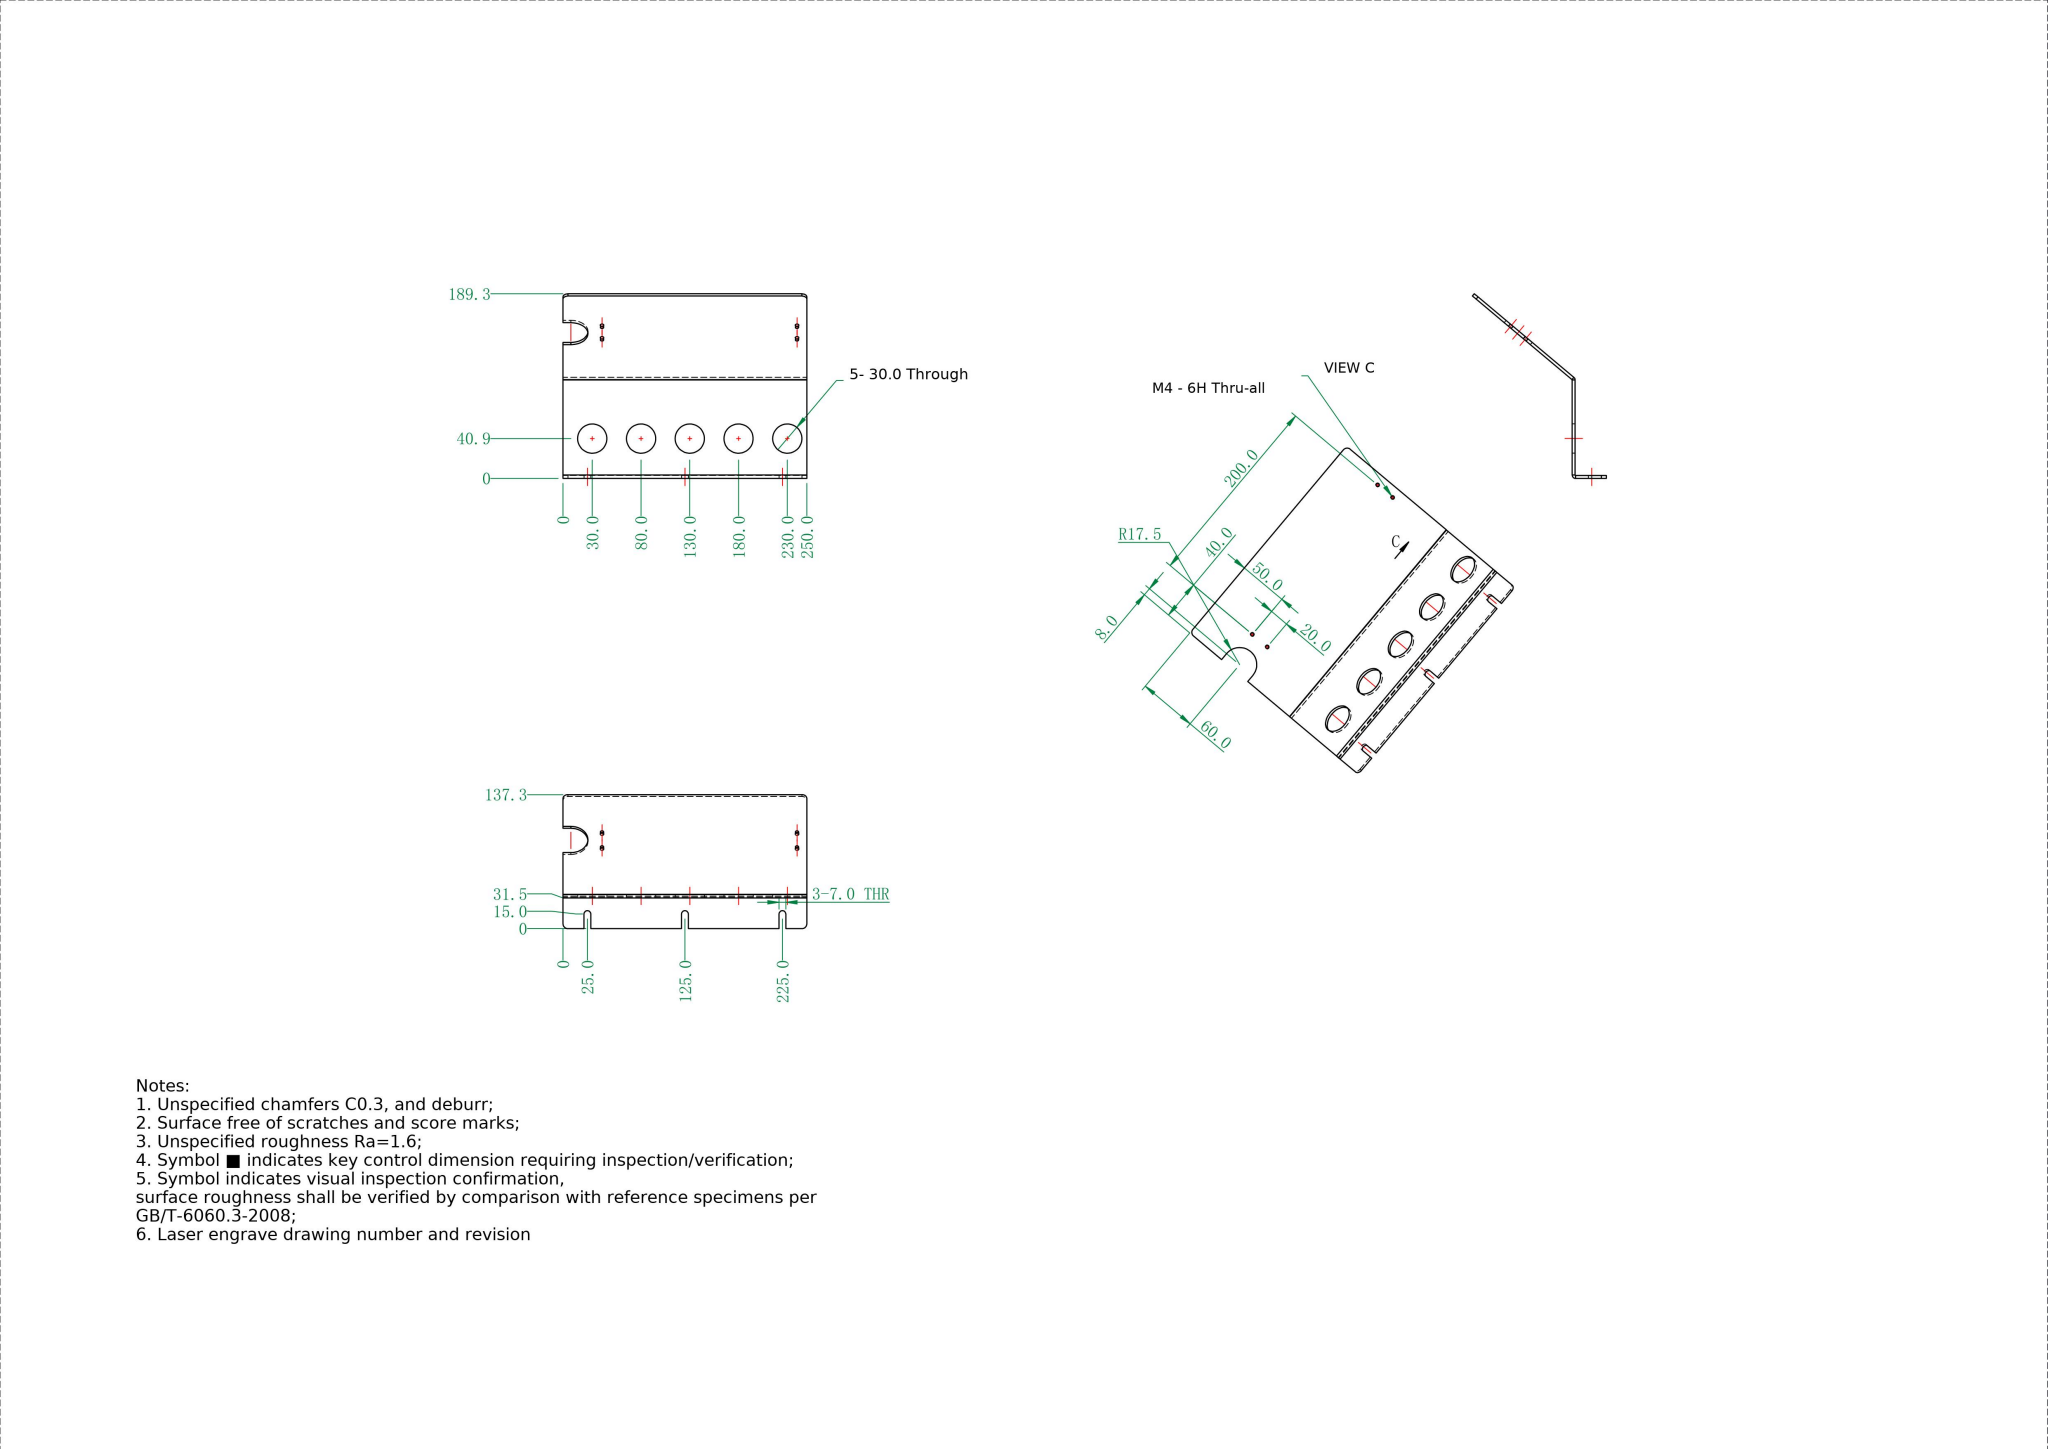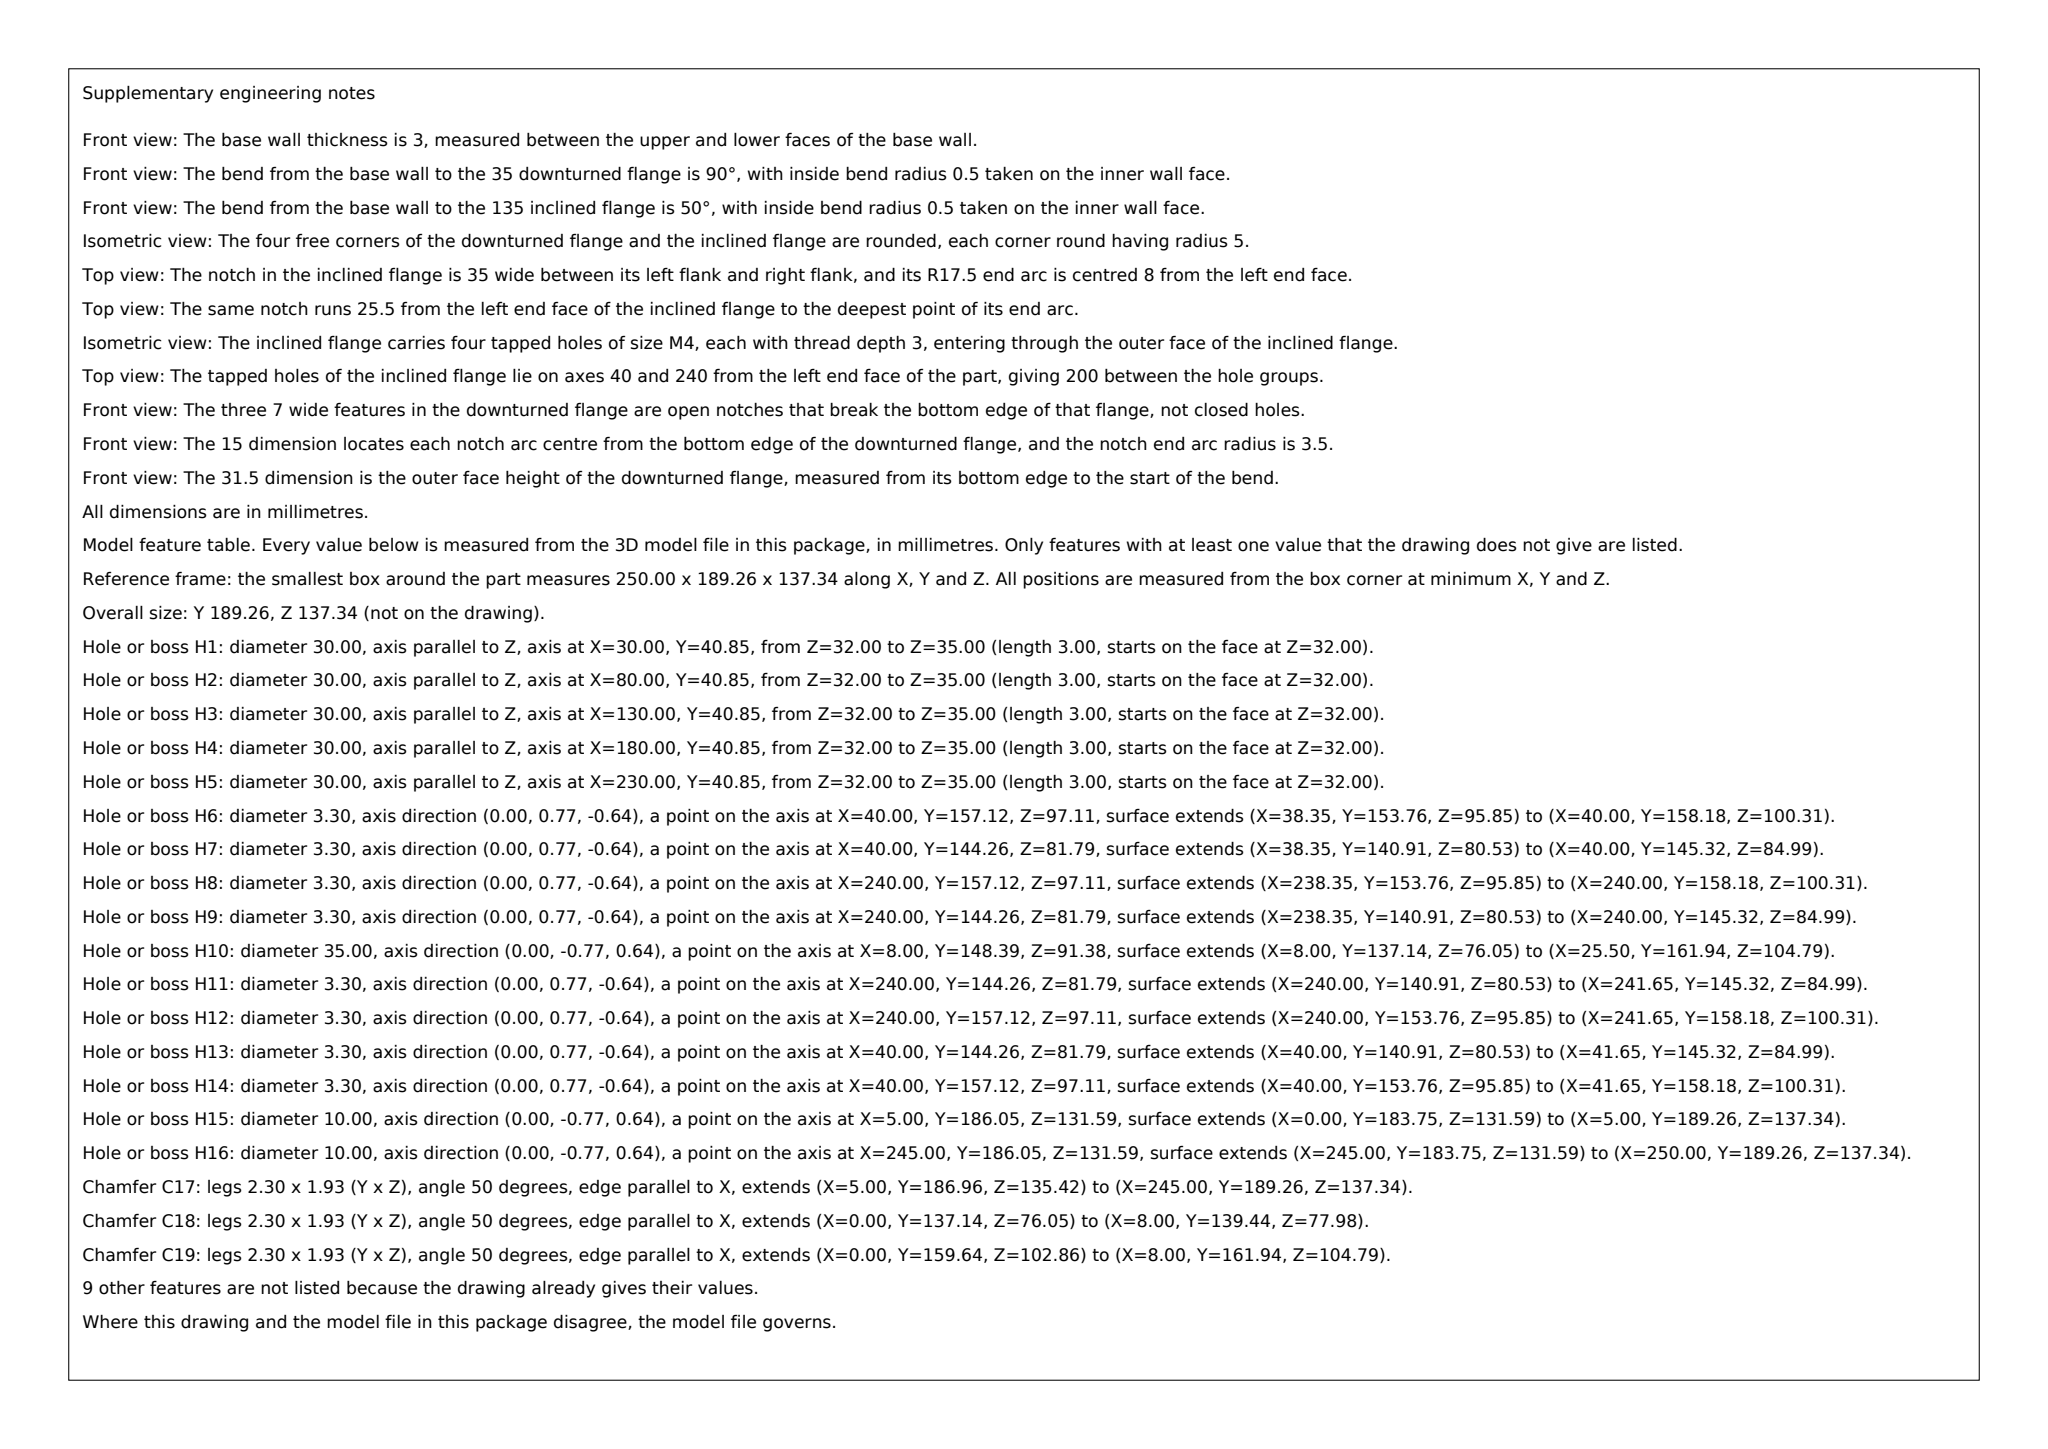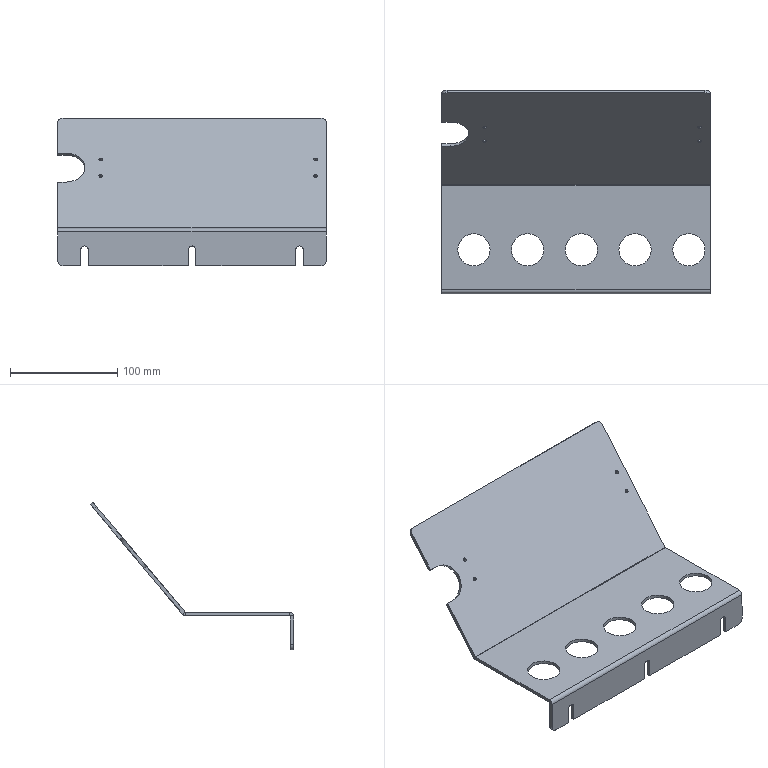Part | SolidWorks | mm | 1 solid | 63 faces | box 250 x 189.26 x 137.34 mm | volume 186158 mm3 | cylinder 33 | plane 30 | commonest cylinder face diameters 30 x10 7 x8 3.3 x8 10 x4 1 x2 35 x1